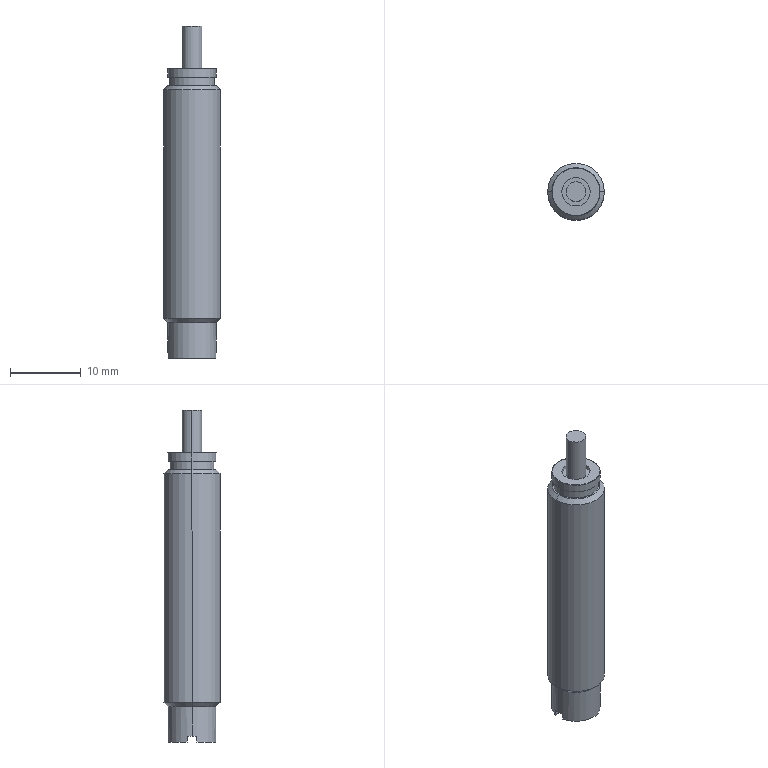Component | SolidWorks | RB0806-1_RB0806-1-1 | 1 solid | 29 faces | box 8 x 8 x 46.8 mm | volume 1959 mm3 | cylinder 12 | plane 11 | cone 4 | spline 2 | commonest cylinder face diameters 6.8 x4 8 x2 6.3 x2 4 x2 2.8 x2
STEP:
#1=COLOUR_RGB('',0.7922,0.8196,0.9333);
#2=FILL_AREA_STYLE_COLOUR('',#1);
#3=FILL_AREA_STYLE('',(#2));
#4=SURFACE_STYLE_FILL_AREA(#3);
#5=SURFACE_SIDE_STYLE('',(#4));
#6=SURFACE_STYLE_USAGE(.BOTH.,#5);
#7=PRESENTATION_STYLE_ASSIGNMENT((#6));
#8=CARTESIAN_POINT('',(-0.9725,1.668,-0.2362));
#9=VERTEX_POINT('',#8);
#10=CARTESIAN_POINT('',(-0.7087,1.668,-0.2362));
#11=VERTEX_POINT('',#10);
#12=CARTESIAN_POINT('',(-0.9725,1.668,-0.2362));
#13=CARTESIAN_POINT('',(-0.9725,1.932,-0.2362));
#14=CARTESIAN_POINT('',(-0.7087,1.932,-0.2362));
#15=CARTESIAN_POINT('',(-0.7087,1.668,-0.2362));
#16=(BOUNDED_CURVE()B_SPLINE_CURVE(3,(#12,#13,#14,#15),.UNSPECIFIED.,.F.,.T.)B_SPLINE_CURVE_WITH_KNOTS((4,4),(0.,1.),.UNSPECIFIED.)CURVE()GEOMETRIC_REPRESENTATION_ITEM()RATIONAL_B_SPLINE_CURVE((1.,0.3333,0.3333,1.))REPRESENTATION_ITEM(''));
#17=EDGE_CURVE('',#9,#11,#16,.T.);
#18=ORIENTED_EDGE('',*,*,#17,.T.);
#19=CARTESIAN_POINT('',(-0.7067,1.668,-0.2382));
#20=VERTEX_POINT('',#19);
#21=CARTESIAN_POINT('',(-0.7087,1.668,-0.2382));
#22=DIRECTION('',(0.,1.,-0.));
#23=DIRECTION('',(1.,0.,0.));
#24=AXIS2_PLACEMENT_3D('',#21,#22,#23);
#25=CIRCLE('',#24,0.001969);
#26=EDGE_CURVE('',#11,#20,#25,.T.);
#27=ORIENTED_EDGE('',*,*,#26,.T.);
#28=CARTESIAN_POINT('',(-0.9744,1.668,-0.2382));
#29=VERTEX_POINT('',#28);
#30=CARTESIAN_POINT('',(-0.8406,1.668,-0.2382));
#31=DIRECTION('',(0.,-0.,-1.));
#32=DIRECTION('',(1.,0.,0.));
#33=AXIS2_PLACEMENT_3D('',#30,#31,#32);
#34=CIRCLE('',#33,0.1339);
#35=EDGE_CURVE('',#29,#20,#34,.T.);
#36=ORIENTED_EDGE('',*,*,#35,.F.);
#37=CARTESIAN_POINT('',(-0.9725,1.668,-0.2382));
#38=DIRECTION('',(-0.,-1.,0.));
#39=DIRECTION('',(-1.,0.,0.));
#40=AXIS2_PLACEMENT_3D('',#37,#38,#39);
#41=CIRCLE('',#40,0.001969);
#42=EDGE_CURVE('',#9,#29,#41,.T.);
#43=ORIENTED_EDGE('',*,*,#42,.F.);
#44=EDGE_LOOP('',(#18,#27,#36,#43));
#45=FACE_OUTER_BOUND('',#44,.T.);
#46=CARTESIAN_POINT('',(-0.7087,1.668,-0.2362));
#47=CARTESIAN_POINT('',(-0.7087,1.932,-0.2362));
#48=CARTESIAN_POINT('',(-0.9725,1.932,-0.2362));
#49=CARTESIAN_POINT('',(-0.9725,1.668,-0.2362));
#50=CARTESIAN_POINT('',(-0.7075,1.668,-0.2362));
#51=CARTESIAN_POINT('',(-0.7075,1.934,-0.2362));
#52=CARTESIAN_POINT('',(-0.9736,1.934,-0.2362));
#53=CARTESIAN_POINT('',(-0.9736,1.668,-0.2362));
#54=CARTESIAN_POINT('',(-0.7067,1.668,-0.237));
#55=CARTESIAN_POINT('',(-0.7067,1.936,-0.237));
#56=CARTESIAN_POINT('',(-0.9744,1.936,-0.237));
#57=CARTESIAN_POINT('',(-0.9744,1.668,-0.237));
#58=CARTESIAN_POINT('',(-0.7067,1.668,-0.2382));
#59=CARTESIAN_POINT('',(-0.7067,1.936,-0.2382));
#60=CARTESIAN_POINT('',(-0.9744,1.936,-0.2382));
#61=CARTESIAN_POINT('',(-0.9744,1.668,-0.2382));
#62=(BOUNDED_SURFACE()B_SPLINE_SURFACE(3,3,((#46,#47,#48,#49),(#50,#51,#52,#53),(#54,#55,#56,#57),(#58,#59,#60,#61)),.UNSPECIFIED.,.F.,.F.,.F.)B_SPLINE_SURFACE_WITH_KNOTS((4,4),(4,4),(0.,1.),(0.,1.),.UNSPECIFIED.)GEOMETRIC_REPRESENTATION_ITEM()RATIONAL_B_SPLINE_SURFACE(((1.,0.3333,0.3333,1.),(0.8047,0.2682,0.2682,0.8047),(0.8047,0.2682,0.2682,0.8047),(1.,0.3333,0.3333,1.)))REPRESENTATION_ITEM('')SURFACE());
#63=ADVANCED_FACE('',(#45),#62,.T.);
#64=CARTESIAN_POINT('',(-0.6831,1.668,-0.3549));
#65=VERTEX_POINT('',#64);
#66=CARTESIAN_POINT('',(-0.9981,1.668,-0.3549));
#67=VERTEX_POINT('',#66);
#68=CARTESIAN_POINT('',(-0.8406,1.668,-0.3549));
#69=DIRECTION('',(0.,-0.,-1.));
#70=DIRECTION('',(1.,0.,0.));
#71=AXIS2_PLACEMENT_3D('',#68,#69,#70);
#72=CIRCLE('',#71,0.1575);
#73=EDGE_CURVE('',#65,#67,#72,.T.);
#74=ORIENTED_EDGE('',*,*,#73,.T.);
#75=CARTESIAN_POINT('',(-0.9981,1.668,-1.622));
#76=VERTEX_POINT('',#75);
#77=CARTESIAN_POINT('',(-0.9981,1.668,-0.9882));
#78=DIRECTION('',(0.,-0.,-1.));
#79=VECTOR('',#78,39.37);
#80=LINE('',#77,#79);
#81=EDGE_CURVE('',#67,#76,#80,.T.);
#82=ORIENTED_EDGE('',*,*,#81,.T.);
#83=CARTESIAN_POINT('',(-0.6831,1.668,-1.622));
#84=VERTEX_POINT('',#83);
#85=CARTESIAN_POINT('',(-0.8406,1.668,-1.622));
#86=DIRECTION('',(-0.,0.,1.));
#87=DIRECTION('',(1.,0.,0.));
#88=AXIS2_PLACEMENT_3D('',#85,#86,#87);
#89=CIRCLE('',#88,0.1575);
#90=EDGE_CURVE('',#76,#84,#89,.T.);
#91=ORIENTED_EDGE('',*,*,#90,.T.);
#92=CARTESIAN_POINT('',(-0.6831,1.668,-0.9882));
#93=DIRECTION('',(0.,-0.,-1.));
#94=VECTOR('',#93,39.37);
#95=LINE('',#92,#94);
#96=EDGE_CURVE('',#65,#84,#95,.T.);
#97=ORIENTED_EDGE('',*,*,#96,.F.);
#98=EDGE_LOOP('',(#74,#82,#91,#97));
#99=FACE_OUTER_BOUND('',#98,.T.);
#100=CARTESIAN_POINT('',(-0.8406,1.668,-0.9882));
#101=DIRECTION('',(0.,-0.,-1.));
#102=DIRECTION('',(1.,0.,0.));
#103=AXIS2_PLACEMENT_3D('',#100,#101,#102);
#104=CYLINDRICAL_SURFACE('',#103,0.1575);
#105=ADVANCED_FACE('',(#99),#104,.T.);
#106=CARTESIAN_POINT('',(-0.7073,1.668,-0.3307));
#107=VERTEX_POINT('',#106);
#108=CARTESIAN_POINT('',(-0.9739,1.668,-0.3307));
#109=VERTEX_POINT('',#108);
#110=CARTESIAN_POINT('',(-0.8406,1.668,-0.3307));
#111=DIRECTION('',(0.,-0.,-1.));
#112=DIRECTION('',(1.,0.,0.));
#113=AXIS2_PLACEMENT_3D('',#110,#111,#112);
#114=CIRCLE('',#113,0.1333);
#115=EDGE_CURVE('',#107,#109,#114,.T.);
#116=ORIENTED_EDGE('',*,*,#115,.T.);
#117=CARTESIAN_POINT('',(-0.9981,1.668,-0.3549));
#118=DIRECTION('',(-0.7071,-0.,-0.7071));
#119=VECTOR('',#118,39.37);
#120=LINE('',#117,#119);
#121=EDGE_CURVE('',#109,#67,#120,.T.);
#122=ORIENTED_EDGE('',*,*,#121,.T.);
#123=ORIENTED_EDGE('',*,*,#73,.F.);
#124=CARTESIAN_POINT('',(-0.6831,1.668,-0.3549));
#125=DIRECTION('',(0.7071,-0.,-0.7071));
#126=VECTOR('',#125,39.37);
#127=LINE('',#124,#126);
#128=EDGE_CURVE('',#107,#65,#127,.T.);
#129=ORIENTED_EDGE('',*,*,#128,.F.);
#130=EDGE_LOOP('',(#116,#122,#123,#129));
#131=FACE_OUTER_BOUND('',#130,.T.);
#132=CARTESIAN_POINT('',(-0.8406,1.668,-0.3549));
#133=DIRECTION('',(0.,-0.,-1.));
#134=DIRECTION('',(1.,0.,0.));
#135=AXIS2_PLACEMENT_3D('',#132,#133,#134);
#136=CONICAL_SURFACE('',#135,0.1575,0.7854);
#137=ADVANCED_FACE('',(#131),#136,.T.);
#138=CARTESIAN_POINT('',(-0.9739,1.668,-1.646));
#139=VERTEX_POINT('',#138);
#140=CARTESIAN_POINT('',(-0.7073,1.668,-1.646));
#141=VERTEX_POINT('',#140);
#142=CARTESIAN_POINT('',(-0.8406,1.668,-1.646));
#143=DIRECTION('',(-0.,0.,1.));
#144=DIRECTION('',(-1.,0.,0.));
#145=AXIS2_PLACEMENT_3D('',#142,#143,#144);
#146=CIRCLE('',#145,0.1333);
#147=EDGE_CURVE('',#139,#141,#146,.T.);
#148=ORIENTED_EDGE('',*,*,#147,.T.);
#149=CARTESIAN_POINT('',(-0.6831,1.668,-1.622));
#150=DIRECTION('',(0.7071,-0.,0.7071));
#151=VECTOR('',#150,39.37);
#152=LINE('',#149,#151);
#153=EDGE_CURVE('',#141,#84,#152,.T.);
#154=ORIENTED_EDGE('',*,*,#153,.T.);
#155=ORIENTED_EDGE('',*,*,#90,.F.);
#156=CARTESIAN_POINT('',(-0.9981,1.668,-1.622));
#157=DIRECTION('',(-0.7071,0.,0.7071));
#158=VECTOR('',#157,39.37);
#159=LINE('',#156,#158);
#160=EDGE_CURVE('',#139,#76,#159,.T.);
#161=ORIENTED_EDGE('',*,*,#160,.F.);
#162=EDGE_LOOP('',(#148,#154,#155,#161));
#163=FACE_OUTER_BOUND('',#162,.T.);
#164=CARTESIAN_POINT('',(-0.8406,1.668,-1.622));
#165=DIRECTION('',(-0.,0.,1.));
#166=DIRECTION('',(-1.,0.,0.));
#167=AXIS2_PLACEMENT_3D('',#164,#165,#166);
#168=CONICAL_SURFACE('',#167,0.1575,0.7854);
#169=ADVANCED_FACE('',(#163),#168,.T.);
#170=CARTESIAN_POINT('',(-0.7166,1.668,-0.2835));
#171=VERTEX_POINT('',#170);
#172=CARTESIAN_POINT('',(-0.9646,1.668,-0.2835));
#173=VERTEX_POINT('',#172);
#174=CARTESIAN_POINT('',(-0.8406,1.668,-0.2835));
#175=DIRECTION('',(0.,-0.,-1.));
#176=DIRECTION('',(1.,0.,0.));
#177=AXIS2_PLACEMENT_3D('',#174,#175,#176);
#178=CIRCLE('',#177,0.124);
#179=EDGE_CURVE('',#171,#173,#178,.T.);
#180=ORIENTED_EDGE('',*,*,#179,.T.);
#181=CARTESIAN_POINT('',(-0.9646,1.668,-0.3307));
#182=VERTEX_POINT('',#181);
#183=CARTESIAN_POINT('',(-0.9646,1.668,-0.3071));
#184=DIRECTION('',(0.,-0.,-1.));
#185=VECTOR('',#184,39.37);
#186=LINE('',#183,#185);
#187=EDGE_CURVE('',#173,#182,#186,.T.);
#188=ORIENTED_EDGE('',*,*,#187,.T.);
#189=CARTESIAN_POINT('',(-0.7166,1.668,-0.3307));
#190=VERTEX_POINT('',#189);
#191=CARTESIAN_POINT('',(-0.8406,1.668,-0.3307));
#192=DIRECTION('',(0.,-0.,-1.));
#193=DIRECTION('',(1.,0.,0.));
#194=AXIS2_PLACEMENT_3D('',#191,#192,#193);
#195=CIRCLE('',#194,0.124);
#196=EDGE_CURVE('',#190,#182,#195,.T.);
#197=ORIENTED_EDGE('',*,*,#196,.F.);
#198=CARTESIAN_POINT('',(-0.7166,1.668,-0.3071));
#199=DIRECTION('',(0.,-0.,-1.));
#200=VECTOR('',#199,39.37);
#201=LINE('',#198,#200);
#202=EDGE_CURVE('',#171,#190,#201,.T.);
#203=ORIENTED_EDGE('',*,*,#202,.F.);
#204=EDGE_LOOP('',(#180,#188,#197,#203));
#205=FACE_OUTER_BOUND('',#204,.T.);
#206=CARTESIAN_POINT('',(-0.8406,1.668,-0.3071));
#207=DIRECTION('',(0.,-0.,-1.));
#208=DIRECTION('',(1.,0.,0.));
#209=AXIS2_PLACEMENT_3D('',#206,#207,#208);
#210=CYLINDRICAL_SURFACE('',#209,0.124);
#211=ADVANCED_FACE('',(#205),#210,.T.);
#212=CARTESIAN_POINT('',(-0.9744,1.668,-1.646));
#213=VERTEX_POINT('',#212);
#214=CARTESIAN_POINT('',(-0.7067,1.668,-1.646));
#215=VERTEX_POINT('',#214);
#216=CARTESIAN_POINT('',(-0.8406,1.668,-1.646));
#217=DIRECTION('',(-0.,0.,1.));
#218=DIRECTION('',(1.,0.,0.));
#219=AXIS2_PLACEMENT_3D('',#216,#217,#218);
#220=CIRCLE('',#219,0.1339);
#221=EDGE_CURVE('',#213,#215,#220,.T.);
#222=ORIENTED_EDGE('',*,*,#221,.F.);
#223=CARTESIAN_POINT('',(-0.9744,1.668,-1.811));
#224=VERTEX_POINT('',#223);
#225=CARTESIAN_POINT('',(-0.9744,1.668,-1.744));
#226=DIRECTION('',(0.,-0.,-1.));
#227=VECTOR('',#226,39.37);
#228=LINE('',#225,#227);
#229=EDGE_CURVE('',#213,#224,#228,.T.);
#230=ORIENTED_EDGE('',*,*,#229,.T.);
#231=CARTESIAN_POINT('',(-0.9716,1.64,-1.811));
#232=VERTEX_POINT('',#231);
#233=CARTESIAN_POINT('',(-0.8406,1.668,-1.811));
#234=DIRECTION('',(-0.,0.,1.));
#235=DIRECTION('',(1.,0.,0.));
#236=AXIS2_PLACEMENT_3D('',#233,#234,#235);
#237=CIRCLE('',#236,0.1339);
#238=EDGE_CURVE('',#224,#232,#237,.T.);
#239=ORIENTED_EDGE('',*,*,#238,.T.);
#240=CARTESIAN_POINT('',(-0.9716,1.64,-1.843));
#241=VERTEX_POINT('',#240);
#242=CARTESIAN_POINT('',(-0.9716,1.64,-1.843));
#243=DIRECTION('',(0.,-0.,-1.));
#244=VECTOR('',#243,39.37);
#245=LINE('',#242,#244);
#246=EDGE_CURVE('',#232,#241,#245,.T.);
#247=ORIENTED_EDGE('',*,*,#246,.T.);
#248=CARTESIAN_POINT('',(-0.7096,1.64,-1.843));
#249=VERTEX_POINT('',#248);
#250=CARTESIAN_POINT('',(-0.8406,1.668,-1.843));
#251=DIRECTION('',(-0.,0.,1.));
#252=DIRECTION('',(1.,0.,0.));
#253=AXIS2_PLACEMENT_3D('',#250,#251,#252);
#254=CIRCLE('',#253,0.1339);
#255=EDGE_CURVE('',#241,#249,#254,.T.);
#256=ORIENTED_EDGE('',*,*,#255,.T.);
#257=CARTESIAN_POINT('',(-0.7096,1.64,-1.811));
#258=VERTEX_POINT('',#257);
#259=CARTESIAN_POINT('',(-0.7096,1.64,-1.843));
#260=DIRECTION('',(-0.,0.,1.));
#261=VECTOR('',#260,39.37);
#262=LINE('',#259,#261);
#263=EDGE_CURVE('',#249,#258,#262,.T.);
#264=ORIENTED_EDGE('',*,*,#263,.T.);
#265=CARTESIAN_POINT('',(-0.7067,1.668,-1.811));
#266=VERTEX_POINT('',#265);
#267=CARTESIAN_POINT('',(-0.8406,1.668,-1.811));
#268=DIRECTION('',(-0.,0.,1.));
#269=DIRECTION('',(1.,0.,0.));
#270=AXIS2_PLACEMENT_3D('',#267,#268,#269);
#271=CIRCLE('',#270,0.1339);
#272=EDGE_CURVE('',#258,#266,#271,.T.);
#273=ORIENTED_EDGE('',*,*,#272,.T.);
#274=CARTESIAN_POINT('',(-0.7067,1.668,-1.744));
#275=DIRECTION('',(0.,-0.,-1.));
#276=VECTOR('',#275,39.37);
#277=LINE('',#274,#276);
#278=EDGE_CURVE('',#215,#266,#277,.T.);
#279=ORIENTED_EDGE('',*,*,#278,.F.);
#280=EDGE_LOOP('',(#222,#230,#239,#247,#256,#264,#273,#279));
#281=FACE_OUTER_BOUND('',#280,.T.);
#282=CARTESIAN_POINT('',(-0.8406,1.668,-1.744));
#283=DIRECTION('',(0.,-0.,-1.));
#284=DIRECTION('',(1.,0.,0.));
#285=AXIS2_PLACEMENT_3D('',#282,#283,#284);
#286=CYLINDRICAL_SURFACE('',#285,0.1339);
#287=ADVANCED_FACE('',(#281),#286,.T.);
#288=CARTESIAN_POINT('',(-0.8406,1.668,-0.2382));
#289=DIRECTION('',(0.,-0.,-1.));
#290=DIRECTION('',(1.,0.,0.));
#291=AXIS2_PLACEMENT_3D('',#288,#289,#290);
#292=CIRCLE('',#291,0.1339);
#293=EDGE_CURVE('',#20,#29,#292,.T.);
#294=ORIENTED_EDGE('',*,*,#293,.T.);
#295=CARTESIAN_POINT('',(-0.9744,1.668,-0.2835));
#296=VERTEX_POINT('',#295);
#297=CARTESIAN_POINT('',(-0.9744,1.668,-0.2608));
#298=DIRECTION('',(0.,-0.,-1.));
#299=VECTOR('',#298,39.37);
#300=LINE('',#297,#299);
#301=EDGE_CURVE('',#29,#296,#300,.T.);
#302=ORIENTED_EDGE('',*,*,#301,.T.);
#303=CARTESIAN_POINT('',(-0.7067,1.668,-0.2835));
#304=VERTEX_POINT('',#303);
#305=CARTESIAN_POINT('',(-0.8406,1.668,-0.2835));
#306=DIRECTION('',(0.,-0.,-1.));
#307=DIRECTION('',(1.,0.,0.));
#308=AXIS2_PLACEMENT_3D('',#305,#306,#307);
#309=CIRCLE('',#308,0.1339);
#310=EDGE_CURVE('',#304,#296,#309,.T.);
#311=ORIENTED_EDGE('',*,*,#310,.F.);
#312=CARTESIAN_POINT('',(-0.7067,1.668,-0.2608));
#313=DIRECTION('',(0.,-0.,-1.));
#314=VECTOR('',#313,39.37);
#315=LINE('',#312,#314);
#316=EDGE_CURVE('',#20,#304,#315,.T.);
#317=ORIENTED_EDGE('',*,*,#316,.F.);
#318=EDGE_LOOP('',(#294,#302,#311,#317));
#319=FACE_OUTER_BOUND('',#318,.T.);
#320=CARTESIAN_POINT('',(-0.8406,1.668,-0.2608));
#321=DIRECTION('',(0.,-0.,-1.));
#322=DIRECTION('',(1.,0.,0.));
#323=AXIS2_PLACEMENT_3D('',#320,#321,#322);
#324=CYLINDRICAL_SURFACE('',#323,0.1339);
#325=ADVANCED_FACE('',(#319),#324,.T.);
#326=CARTESIAN_POINT('',(-0.7618,1.668,-0.2559));
#327=VERTEX_POINT('',#326);
#328=CARTESIAN_POINT('',(-0.9193,1.668,-0.2559));
#329=VERTEX_POINT('',#328);
#330=CARTESIAN_POINT('',(-0.8406,1.668,-0.2559));
#331=DIRECTION('',(-0.,0.,1.));
#332=DIRECTION('',(-1.,0.,0.));
#333=AXIS2_PLACEMENT_3D('',#330,#331,#332);
#334=CIRCLE('',#333,0.07874);
#335=EDGE_CURVE('',#327,#329,#334,.T.);
#336=ORIENTED_EDGE('',*,*,#335,.F.);
#337=CARTESIAN_POINT('',(-0.7618,1.668,-0.2362));
#338=VERTEX_POINT('',#337);
#339=CARTESIAN_POINT('',(-0.7618,1.668,-0.2362));
#340=DIRECTION('',(-0.,0.,1.));
#341=VECTOR('',#340,39.37);
#342=LINE('',#339,#341);
#343=EDGE_CURVE('',#327,#338,#342,.T.);
#344=ORIENTED_EDGE('',*,*,#343,.T.);
#345=CARTESIAN_POINT('',(-0.9193,1.668,-0.2362));
#346=VERTEX_POINT('',#345);
#347=CARTESIAN_POINT('',(-0.8406,1.668,-0.2362));
#348=DIRECTION('',(0.,-0.,-1.));
#349=DIRECTION('',(-1.,0.,0.));
#350=AXIS2_PLACEMENT_3D('',#347,#348,#349);
#351=CIRCLE('',#350,0.07874);
#352=EDGE_CURVE('',#346,#338,#351,.T.);
#353=ORIENTED_EDGE('',*,*,#352,.F.);
#354=CARTESIAN_POINT('',(-0.9193,1.668,-0.2362));
#355=DIRECTION('',(-0.,0.,1.));
#356=VECTOR('',#355,39.37);
#357=LINE('',#354,#356);
#358=EDGE_CURVE('',#329,#346,#357,.T.);
#359=ORIENTED_EDGE('',*,*,#358,.F.);
#360=EDGE_LOOP('',(#336,#344,#353,#359));
#361=FACE_OUTER_BOUND('',#360,.T.);
#362=CARTESIAN_POINT('',(-0.8406,1.668,-0.2362));
#363=DIRECTION('',(-0.,0.,1.));
#364=DIRECTION('',(-1.,0.,0.));
#365=AXIS2_PLACEMENT_3D('',#362,#363,#364);
#366=CYLINDRICAL_SURFACE('',#365,0.07874);
#367=ADVANCED_FACE('',(#361),#366,.F.);
#368=CARTESIAN_POINT('',(-0.7855,1.668,-0.));
#369=VERTEX_POINT('',#368);
#370=CARTESIAN_POINT('',(-0.8957,1.668,-0.));
#371=VERTEX_POINT('',#370);
#372=CARTESIAN_POINT('',(-0.8406,1.668,-0.));
#373=DIRECTION('',(0.,-0.,-1.));
#374=DIRECTION('',(1.,0.,0.));
#375=AXIS2_PLACEMENT_3D('',#372,#373,#374);
#376=CIRCLE('',#375,0.05512);
#377=EDGE_CURVE('',#369,#371,#376,.T.);
#378=ORIENTED_EDGE('',*,*,#377,.T.);
#379=CARTESIAN_POINT('',(-0.8957,1.668,-0.2559));
#380=VERTEX_POINT('',#379);
#381=CARTESIAN_POINT('',(-0.8957,1.668,-0.2362));
#382=DIRECTION('',(0.,-0.,-1.));
#383=VECTOR('',#382,39.37);
#384=LINE('',#381,#383);
#385=EDGE_CURVE('',#371,#380,#384,.T.);
#386=ORIENTED_EDGE('',*,*,#385,.T.);
#387=CARTESIAN_POINT('',(-0.7855,1.668,-0.2559));
#388=VERTEX_POINT('',#387);
#389=CARTESIAN_POINT('',(-0.8406,1.668,-0.2559));
#390=DIRECTION('',(-0.,0.,1.));
#391=DIRECTION('',(1.,0.,0.));
#392=AXIS2_PLACEMENT_3D('',#389,#390,#391);
#393=CIRCLE('',#392,0.05512);
#394=EDGE_CURVE('',#380,#388,#393,.T.);
#395=ORIENTED_EDGE('',*,*,#394,.T.);
#396=CARTESIAN_POINT('',(-0.7855,1.668,-0.2362));
#397=DIRECTION('',(0.,-0.,-1.));
#398=VECTOR('',#397,39.37);
#399=LINE('',#396,#398);
#400=EDGE_CURVE('',#369,#388,#399,.T.);
#401=ORIENTED_EDGE('',*,*,#400,.F.);
#402=EDGE_LOOP('',(#378,#386,#395,#401));
#403=FACE_OUTER_BOUND('',#402,.T.);
#404=CARTESIAN_POINT('',(-0.8406,1.668,-0.2362));
#405=DIRECTION('',(0.,-0.,-1.));
#406=DIRECTION('',(1.,0.,0.));
#407=AXIS2_PLACEMENT_3D('',#404,#405,#406);
#408=CYLINDRICAL_SURFACE('',#407,0.05512);
#409=ADVANCED_FACE('',(#403),#408,.T.);
#410=ORIENTED_EDGE('',*,*,#81,.F.);
#411=CARTESIAN_POINT('',(-0.8406,1.668,-0.3549));
#412=DIRECTION('',(0.,-0.,-1.));
#413=DIRECTION('',(1.,0.,0.));
#414=AXIS2_PLACEMENT_3D('',#411,#412,#413);
#415=CIRCLE('',#414,0.1575);
#416=EDGE_CURVE('',#67,#65,#415,.T.);
#417=ORIENTED_EDGE('',*,*,#416,.T.);
#418=ORIENTED_EDGE('',*,*,#96,.T.);
#419=CARTESIAN_POINT('',(-0.8406,1.668,-1.622));
#420=DIRECTION('',(-0.,0.,1.));
#421=DIRECTION('',(1.,0.,0.));
#422=AXIS2_PLACEMENT_3D('',#419,#420,#421);
#423=CIRCLE('',#422,0.1575);
#424=EDGE_CURVE('',#84,#76,#423,.T.);
#425=ORIENTED_EDGE('',*,*,#424,.T.);
#426=EDGE_LOOP('',(#410,#417,#418,#425));
#427=FACE_OUTER_BOUND('',#426,.T.);
#428=CARTESIAN_POINT('',(-0.8406,1.668,-0.9882));
#429=DIRECTION('',(0.,-0.,-1.));
#430=DIRECTION('',(1.,0.,0.));
#431=AXIS2_PLACEMENT_3D('',#428,#429,#430);
#432=CYLINDRICAL_SURFACE('',#431,0.1575);
#433=ADVANCED_FACE('',(#427),#432,.T.);
#434=ORIENTED_EDGE('',*,*,#121,.F.);
#435=CARTESIAN_POINT('',(-0.8406,1.668,-0.3307));
#436=DIRECTION('',(0.,-0.,-1.));
#437=DIRECTION('',(1.,0.,0.));
#438=AXIS2_PLACEMENT_3D('',#435,#436,#437);
#439=CIRCLE('',#438,0.1333);
#440=EDGE_CURVE('',#109,#107,#439,.T.);
#441=ORIENTED_EDGE('',*,*,#440,.T.);
#442=ORIENTED_EDGE('',*,*,#128,.T.);
#443=ORIENTED_EDGE('',*,*,#416,.F.);
#444=EDGE_LOOP('',(#434,#441,#442,#443));
#445=FACE_OUTER_BOUND('',#444,.T.);
#446=CARTESIAN_POINT('',(-0.8406,1.668,-0.3549));
#447=DIRECTION('',(0.,-0.,-1.));
#448=DIRECTION('',(1.,0.,0.));
#449=AXIS2_PLACEMENT_3D('',#446,#447,#448);
#450=CONICAL_SURFACE('',#449,0.1575,0.7854);
#451=ADVANCED_FACE('',(#445),#450,.T.);
#452=ORIENTED_EDGE('',*,*,#153,.F.);
#453=CARTESIAN_POINT('',(-0.8406,1.668,-1.646));
#454=DIRECTION('',(-0.,0.,1.));
#455=DIRECTION('',(-1.,0.,0.));
#456=AXIS2_PLACEMENT_3D('',#453,#454,#455);
#457=CIRCLE('',#456,0.1333);
#458=EDGE_CURVE('',#141,#139,#457,.T.);
#459=ORIENTED_EDGE('',*,*,#458,.T.);
#460=ORIENTED_EDGE('',*,*,#160,.T.);
#461=ORIENTED_EDGE('',*,*,#424,.F.);
#462=EDGE_LOOP('',(#452,#459,#460,#461));
#463=FACE_OUTER_BOUND('',#462,.T.);
#464=CARTESIAN_POINT('',(-0.8406,1.668,-1.622));
#465=DIRECTION('',(-0.,0.,1.));
#466=DIRECTION('',(-1.,0.,0.));
#467=AXIS2_PLACEMENT_3D('',#464,#465,#466);
#468=CONICAL_SURFACE('',#467,0.1575,0.7854);
#469=ADVANCED_FACE('',(#463),#468,.T.);
#470=ORIENTED_EDGE('',*,*,#115,.F.);
#471=ORIENTED_EDGE('',*,*,#440,.F.);
#472=EDGE_LOOP('',(#470,#471));
#473=FACE_OUTER_BOUND('',#472,.T.);
#474=ORIENTED_EDGE('',*,*,#196,.T.);
#475=CARTESIAN_POINT('',(-0.8406,1.668,-0.3307));
#476=DIRECTION('',(0.,-0.,-1.));
#477=DIRECTION('',(1.,0.,0.));
#478=AXIS2_PLACEMENT_3D('',#475,#476,#477);
#479=CIRCLE('',#478,0.124);
#480=EDGE_CURVE('',#182,#190,#479,.T.);
#481=ORIENTED_EDGE('',*,*,#480,.T.);
#482=EDGE_LOOP('',(#474,#481));
#483=FACE_BOUND('',#482,.T.);
#484=CARTESIAN_POINT('',(-0.8406,1.539,-0.3307));
#485=DIRECTION('',(-0.,0.,1.));
#486=DIRECTION('',(-1.,0.,-0.));
#487=AXIS2_PLACEMENT_3D('',#484,#485,#486);
#488=PLANE('',#487);
#489=ADVANCED_FACE('',(#473,#483),#488,.T.);
#490=CARTESIAN_POINT('',(-0.8406,1.668,-1.646));
#491=DIRECTION('',(-0.,0.,1.));
#492=DIRECTION('',(1.,0.,0.));
#493=AXIS2_PLACEMENT_3D('',#490,#491,#492);
#494=CIRCLE('',#493,0.1339);
#495=EDGE_CURVE('',#215,#213,#494,.T.);
#496=ORIENTED_EDGE('',*,*,#495,.T.);
#497=ORIENTED_EDGE('',*,*,#221,.T.);
#498=EDGE_LOOP('',(#496,#497));
#499=FACE_OUTER_BOUND('',#498,.T.);
#500=ORIENTED_EDGE('',*,*,#147,.F.);
#501=ORIENTED_EDGE('',*,*,#458,.F.);
#502=EDGE_LOOP('',(#500,#501));
#503=FACE_BOUND('',#502,.T.);
#504=CARTESIAN_POINT('',(-0.8406,1.534,-1.646));
#505=DIRECTION('',(-0.,0.,1.));
#506=DIRECTION('',(-1.,0.,-0.));
#507=AXIS2_PLACEMENT_3D('',#504,#505,#506);
#508=PLANE('',#507);
#509=ADVANCED_FACE('',(#499,#503),#508,.T.);
#510=ORIENTED_EDGE('',*,*,#187,.F.);
#511=CARTESIAN_POINT('',(-0.8406,1.668,-0.2835));
#512=DIRECTION('',(0.,-0.,-1.));
#513=DIRECTION('',(1.,0.,0.));
#514=AXIS2_PLACEMENT_3D('',#511,#512,#513);
#515=CIRCLE('',#514,0.124);
#516=EDGE_CURVE('',#173,#171,#515,.T.);
#517=ORIENTED_EDGE('',*,*,#516,.T.);
#518=ORIENTED_EDGE('',*,*,#202,.T.);
#519=ORIENTED_EDGE('',*,*,#480,.F.);
#520=EDGE_LOOP('',(#510,#517,#518,#519));
#521=FACE_OUTER_BOUND('',#520,.T.);
#522=CARTESIAN_POINT('',(-0.8406,1.668,-0.3071));
#523=DIRECTION('',(0.,-0.,-1.));
#524=DIRECTION('',(1.,0.,0.));
#525=AXIS2_PLACEMENT_3D('',#522,#523,#524);
#526=CYLINDRICAL_SURFACE('',#525,0.124);
#527=ADVANCED_FACE('',(#521),#526,.T.);
#528=ORIENTED_EDGE('',*,*,#229,.F.);
#529=ORIENTED_EDGE('',*,*,#495,.F.);
#530=ORIENTED_EDGE('',*,*,#278,.T.);
#531=CARTESIAN_POINT('',(-0.7096,1.695,-1.811));
#532=VERTEX_POINT('',#531);
#533=CARTESIAN_POINT('',(-0.8406,1.668,-1.811));
#534=DIRECTION('',(-0.,0.,1.));
#535=DIRECTION('',(1.,0.,0.));
#536=AXIS2_PLACEMENT_3D('',#533,#534,#535);
#537=CIRCLE('',#536,0.1339);
#538=EDGE_CURVE('',#266,#532,#537,.T.);
#539=ORIENTED_EDGE('',*,*,#538,.T.);
#540=CARTESIAN_POINT('',(-0.7096,1.695,-1.843));
#541=VERTEX_POINT('',#540);
#542=CARTESIAN_POINT('',(-0.7096,1.695,-1.811));
#543=DIRECTION('',(0.,-0.,-1.));
#544=VECTOR('',#543,39.37);
#545=LINE('',#542,#544);
#546=EDGE_CURVE('',#532,#541,#545,.T.);
#547=ORIENTED_EDGE('',*,*,#546,.T.);
#548=CARTESIAN_POINT('',(-0.9716,1.695,-1.843));
#549=VERTEX_POINT('',#548);
#550=CARTESIAN_POINT('',(-0.8406,1.668,-1.843));
#551=DIRECTION('',(-0.,0.,1.));
#552=DIRECTION('',(1.,0.,0.));
#553=AXIS2_PLACEMENT_3D('',#550,#551,#552);
#554=CIRCLE('',#553,0.1339);
#555=EDGE_CURVE('',#541,#549,#554,.T.);
#556=ORIENTED_EDGE('',*,*,#555,.T.);
#557=CARTESIAN_POINT('',(-0.9716,1.695,-1.811));
#558=VERTEX_POINT('',#557);
#559=CARTESIAN_POINT('',(-0.9716,1.695,-1.811));
#560=DIRECTION('',(-0.,0.,1.));
#561=VECTOR('',#560,39.37);
#562=LINE('',#559,#561);
#563=EDGE_CURVE('',#549,#558,#562,.T.);
#564=ORIENTED_EDGE('',*,*,#563,.T.);
#565=CARTESIAN_POINT('',(-0.8406,1.668,-1.811));
#566=DIRECTION('',(-0.,0.,1.));
#567=DIRECTION('',(1.,0.,0.));
#568=AXIS2_PLACEMENT_3D('',#565,#566,#567);
#569=CIRCLE('',#568,0.1339);
#570=EDGE_CURVE('',#558,#224,#569,.T.);
#571=ORIENTED_EDGE('',*,*,#570,.T.);
#572=EDGE_LOOP('',(#528,#529,#530,#539,#547,#556,#564,#571));
#573=FACE_OUTER_BOUND('',#572,.T.);
#574=CARTESIAN_POINT('',(-0.8406,1.668,-1.744));
#575=DIRECTION('',(0.,-0.,-1.));
#576=DIRECTION('',(1.,0.,0.));
#577=AXIS2_PLACEMENT_3D('',#574,#575,#576);
#578=CYLINDRICAL_SURFACE('',#577,0.1339);
#579=ADVANCED_FACE('',(#573),#578,.T.);
#580=ORIENTED_EDGE('',*,*,#179,.F.);
#581=ORIENTED_EDGE('',*,*,#516,.F.);
#582=EDGE_LOOP('',(#580,#581));
#583=FACE_BOUND('',#582,.T.);
#584=ORIENTED_EDGE('',*,*,#310,.T.);
#585=CARTESIAN_POINT('',(-0.8406,1.668,-0.2835));
#586=DIRECTION('',(0.,-0.,-1.));
#587=DIRECTION('',(1.,0.,0.));
#588=AXIS2_PLACEMENT_3D('',#585,#586,#587);
#589=CIRCLE('',#588,0.1339);
#590=EDGE_CURVE('',#296,#304,#589,.T.);
#591=ORIENTED_EDGE('',*,*,#590,.T.);
#592=EDGE_LOOP('',(#584,#591));
#593=FACE_OUTER_BOUND('',#592,.T.);
#594=CARTESIAN_POINT('',(-0.8406,1.539,-0.2835));
#595=DIRECTION('',(0.,-0.,-1.));
#596=DIRECTION('',(1.,-0.,0.));
#597=AXIS2_PLACEMENT_3D('',#594,#595,#596);
#598=PLANE('',#597);
#599=ADVANCED_FACE('',(#583,#593),#598,.T.);
#600=CARTESIAN_POINT('',(-0.8406,1.64,-1.843));
#601=DIRECTION('',(1.,-0.,0.));
#602=VECTOR('',#601,39.37);
#603=LINE('',#600,#602);
#604=EDGE_CURVE('',#241,#249,#603,.T.);
#605=ORIENTED_EDGE('',*,*,#604,.T.);
#606=ORIENTED_EDGE('',*,*,#255,.F.);
#607=EDGE_LOOP('',(#605,#606));
#608=FACE_OUTER_BOUND('',#607,.T.);
#609=CARTESIAN_POINT('',(-0.8406,1.601,-1.843));
#610=DIRECTION('',(0.,-0.,-1.));
#611=DIRECTION('',(1.,-0.,0.));
#612=AXIS2_PLACEMENT_3D('',#609,#610,#611);
#613=PLANE('',#612);
#614=ADVANCED_FACE('',(#608),#613,.T.);
#615=ORIENTED_EDGE('',*,*,#555,.F.);
#616=CARTESIAN_POINT('',(-0.8406,1.695,-1.843));
#617=DIRECTION('',(-1.,0.,-0.));
#618=VECTOR('',#617,39.37);
#619=LINE('',#616,#618);
#620=EDGE_CURVE('',#541,#549,#619,.T.);
#621=ORIENTED_EDGE('',*,*,#620,.T.);
#622=EDGE_LOOP('',(#615,#621));
#623=FACE_OUTER_BOUND('',#622,.T.);
#624=CARTESIAN_POINT('',(-0.8406,1.601,-1.843));
#625=DIRECTION('',(0.,-0.,-1.));
#626=DIRECTION('',(1.,-0.,0.));
#627=AXIS2_PLACEMENT_3D('',#624,#625,#626);
#628=PLANE('',#627);
#629=ADVANCED_FACE('',(#623),#628,.T.);
#630=ORIENTED_EDGE('',*,*,#301,.F.);
#631=ORIENTED_EDGE('',*,*,#35,.T.);
#632=ORIENTED_EDGE('',*,*,#316,.T.);
#633=ORIENTED_EDGE('',*,*,#590,.F.);
#634=EDGE_LOOP('',(#630,#631,#632,#633));
#635=FACE_OUTER_BOUND('',#634,.T.);
#636=CARTESIAN_POINT('',(-0.8406,1.668,-0.2608));
#637=DIRECTION('',(0.,-0.,-1.));
#638=DIRECTION('',(1.,0.,0.));
#639=AXIS2_PLACEMENT_3D('',#636,#637,#638);
#640=CYLINDRICAL_SURFACE('',#639,0.1339);
#641=ADVANCED_FACE('',(#635),#640,.T.);
#642=CARTESIAN_POINT('',(-1.108,1.64,-1.811));
#643=DIRECTION('',(-1.,0.,-0.));
#644=VECTOR('',#643,39.37);
#645=LINE('',#642,#644);
#646=EDGE_CURVE('',#258,#232,#645,.T.);
#647=ORIENTED_EDGE('',*,*,#646,.F.);
#648=ORIENTED_EDGE('',*,*,#263,.F.);
#649=ORIENTED_EDGE('',*,*,#604,.F.);
#650=ORIENTED_EDGE('',*,*,#246,.F.);
#651=EDGE_LOOP('',(#647,#648,#649,#650));
#652=FACE_OUTER_BOUND('',#651,.T.);
#653=CARTESIAN_POINT('',(-1.108,1.64,-1.843));
#654=DIRECTION('',(-0.,-1.,0.));
#655=DIRECTION('',(-1.,0.,-0.));
#656=AXIS2_PLACEMENT_3D('',#653,#654,#655);
#657=PLANE('',#656);
#658=ADVANCED_FACE('',(#652),#657,.F.);
#659=ORIENTED_EDGE('',*,*,#620,.F.);
#660=ORIENTED_EDGE('',*,*,#546,.F.);
#661=CARTESIAN_POINT('',(-1.108,1.695,-1.811));
#662=DIRECTION('',(1.,-0.,0.));
#663=VECTOR('',#662,39.37);
#664=LINE('',#661,#663);
#665=EDGE_CURVE('',#558,#532,#664,.T.);
#666=ORIENTED_EDGE('',*,*,#665,.F.);
#667=ORIENTED_EDGE('',*,*,#563,.F.);
#668=EDGE_LOOP('',(#659,#660,#666,#667));
#669=FACE_OUTER_BOUND('',#668,.T.);
#670=CARTESIAN_POINT('',(-1.108,1.695,-1.811));
#671=DIRECTION('',(0.,1.,-0.));
#672=DIRECTION('',(1.,-0.,0.));
#673=AXIS2_PLACEMENT_3D('',#670,#671,#672);
#674=PLANE('',#673);
#675=ADVANCED_FACE('',(#669),#674,.F.);
#676=ORIENTED_EDGE('',*,*,#26,.F.);
#677=CARTESIAN_POINT('',(-0.8406,1.536,-0.2362));
#678=VERTEX_POINT('',#677);
#679=CARTESIAN_POINT('',(-0.7087,1.668,-0.2362));
#680=CARTESIAN_POINT('',(-0.7087,1.591,-0.2362));
#681=CARTESIAN_POINT('',(-0.7633,1.536,-0.2362));
#682=CARTESIAN_POINT('',(-0.8406,1.536,-0.2362));
#683=(BOUNDED_CURVE()B_SPLINE_CURVE(3,(#679,#680,#681,#682),.UNSPECIFIED.,.F.,.F.)B_SPLINE_CURVE_WITH_KNOTS((4,4),(0.,1.),.UNSPECIFIED.)CURVE()GEOMETRIC_REPRESENTATION_ITEM()RATIONAL_B_SPLINE_CURVE((1.,0.8047,0.8047,1.))REPRESENTATION_ITEM(''));
#684=EDGE_CURVE('',#11,#678,#683,.T.);
#685=ORIENTED_EDGE('',*,*,#684,.T.);
#686=CARTESIAN_POINT('',(-0.8406,1.536,-0.2362));
#687=CARTESIAN_POINT('',(-0.9178,1.536,-0.2362));
#688=CARTESIAN_POINT('',(-0.9725,1.591,-0.2362));
#689=CARTESIAN_POINT('',(-0.9725,1.668,-0.2362));
#690=(BOUNDED_CURVE()B_SPLINE_CURVE(3,(#686,#687,#688,#689),.UNSPECIFIED.,.F.,.F.)B_SPLINE_CURVE_WITH_KNOTS((4,4),(0.,1.),.UNSPECIFIED.)CURVE()GEOMETRIC_REPRESENTATION_ITEM()RATIONAL_B_SPLINE_CURVE((1.,0.8047,0.8047,1.))REPRESENTATION_ITEM(''));
#691=EDGE_CURVE('',#678,#9,#690,.T.);
#692=ORIENTED_EDGE('',*,*,#691,.T.);
#693=ORIENTED_EDGE('',*,*,#42,.T.);
#694=ORIENTED_EDGE('',*,*,#293,.F.);
#695=EDGE_LOOP('',(#676,#685,#692,#693,#694));
#696=FACE_OUTER_BOUND('',#695,.T.);
#697=CARTESIAN_POINT('',(-0.9725,1.668,-0.2362));
#698=CARTESIAN_POINT('',(-0.9725,1.404,-0.2362));
#699=CARTESIAN_POINT('',(-0.7087,1.404,-0.2362));
#700=CARTESIAN_POINT('',(-0.7087,1.668,-0.2362));
#701=CARTESIAN_POINT('',(-0.9736,1.668,-0.2362));
#702=CARTESIAN_POINT('',(-0.9736,1.402,-0.2362));
#703=CARTESIAN_POINT('',(-0.7075,1.402,-0.2362));
#704=CARTESIAN_POINT('',(-0.7075,1.668,-0.2362));
#705=CARTESIAN_POINT('',(-0.9744,1.668,-0.237));
#706=CARTESIAN_POINT('',(-0.9744,1.4,-0.237));
#707=CARTESIAN_POINT('',(-0.7067,1.4,-0.237));
#708=CARTESIAN_POINT('',(-0.7067,1.668,-0.237));
#709=CARTESIAN_POINT('',(-0.9744,1.668,-0.2382));
#710=CARTESIAN_POINT('',(-0.9744,1.4,-0.2382));
#711=CARTESIAN_POINT('',(-0.7067,1.4,-0.2382));
#712=CARTESIAN_POINT('',(-0.7067,1.668,-0.2382));
#713=(BOUNDED_SURFACE()B_SPLINE_SURFACE(3,3,((#697,#698,#699,#700),(#701,#702,#703,#704),(#705,#706,#707,#708),(#709,#710,#711,#712)),.UNSPECIFIED.,.F.,.F.,.F.)B_SPLINE_SURFACE_WITH_KNOTS((4,4),(4,4),(0.,1.),(0.,1.),.UNSPECIFIED.)GEOMETRIC_REPRESENTATION_ITEM()RATIONAL_B_SPLINE_SURFACE(((1.,0.3333,0.3333,1.),(0.8047,0.2682,0.2682,0.8047),(0.8047,0.2682,0.2682,0.8047),(1.,0.3333,0.3333,1.)))REPRESENTATION_ITEM('')SURFACE());
#714=ADVANCED_FACE('',(#696),#713,.T.);
#715=ORIENTED_EDGE('',*,*,#665,.T.);
#716=ORIENTED_EDGE('',*,*,#538,.F.);
#717=ORIENTED_EDGE('',*,*,#272,.F.);
#718=ORIENTED_EDGE('',*,*,#646,.T.);
#719=ORIENTED_EDGE('',*,*,#238,.F.);
#720=ORIENTED_EDGE('',*,*,#570,.F.);
#721=EDGE_LOOP('',(#715,#716,#717,#718,#719,#720));
#722=FACE_OUTER_BOUND('',#721,.T.);
#723=CARTESIAN_POINT('',(-1.108,1.64,-1.811));
#724=DIRECTION('',(-0.,0.,1.));
#725=DIRECTION('',(-1.,0.,-0.));
#726=AXIS2_PLACEMENT_3D('',#723,#724,#725);
#727=PLANE('',#726);
#728=ADVANCED_FACE('',(#722),#727,.F.);
#729=ORIENTED_EDGE('',*,*,#17,.F.);
#730=ORIENTED_EDGE('',*,*,#691,.F.);
#731=ORIENTED_EDGE('',*,*,#684,.F.);
#732=EDGE_LOOP('',(#729,#730,#731));
#733=FACE_OUTER_BOUND('',#732,.T.);
#734=ORIENTED_EDGE('',*,*,#352,.T.);
#735=CARTESIAN_POINT('',(-0.8406,1.668,-0.2362));
#736=DIRECTION('',(0.,-0.,-1.));
#737=DIRECTION('',(-1.,0.,0.));
#738=AXIS2_PLACEMENT_3D('',#735,#736,#737);
#739=CIRCLE('',#738,0.07874);
#740=EDGE_CURVE('',#338,#346,#739,.T.);
#741=ORIENTED_EDGE('',*,*,#740,.T.);
#742=EDGE_LOOP('',(#734,#741));
#743=FACE_BOUND('',#742,.T.);
#744=CARTESIAN_POINT('',(-0.8406,1.602,-0.2362));
#745=DIRECTION('',(-0.,0.,1.));
#746=DIRECTION('',(-1.,0.,-0.));
#747=AXIS2_PLACEMENT_3D('',#744,#745,#746);
#748=PLANE('',#747);
#749=ADVANCED_FACE('',(#733,#743),#748,.T.);
#750=ORIENTED_EDGE('',*,*,#343,.F.);
#751=CARTESIAN_POINT('',(-0.8406,1.668,-0.2559));
#752=DIRECTION('',(-0.,0.,1.));
#753=DIRECTION('',(-1.,0.,0.));
#754=AXIS2_PLACEMENT_3D('',#751,#752,#753);
#755=CIRCLE('',#754,0.07874);
#756=EDGE_CURVE('',#329,#327,#755,.T.);
#757=ORIENTED_EDGE('',*,*,#756,.F.);
#758=ORIENTED_EDGE('',*,*,#358,.T.);
#759=ORIENTED_EDGE('',*,*,#740,.F.);
#760=EDGE_LOOP('',(#750,#757,#758,#759));
#761=FACE_OUTER_BOUND('',#760,.T.);
#762=CARTESIAN_POINT('',(-0.8406,1.668,-0.2362));
#763=DIRECTION('',(-0.,0.,1.));
#764=DIRECTION('',(-1.,0.,0.));
#765=AXIS2_PLACEMENT_3D('',#762,#763,#764);
#766=CYLINDRICAL_SURFACE('',#765,0.07874);
#767=ADVANCED_FACE('',(#761),#766,.F.);
#768=CARTESIAN_POINT('',(-0.8406,1.668,-0.2559));
#769=DIRECTION('',(-0.,0.,1.));
#770=DIRECTION('',(1.,0.,0.));
#771=AXIS2_PLACEMENT_3D('',#768,#769,#770);
#772=CIRCLE('',#771,0.05512);
#773=EDGE_CURVE('',#388,#380,#772,.T.);
#774=ORIENTED_EDGE('',*,*,#773,.F.);
#775=ORIENTED_EDGE('',*,*,#394,.F.);
#776=EDGE_LOOP('',(#774,#775));
#777=FACE_BOUND('',#776,.T.);
#778=ORIENTED_EDGE('',*,*,#756,.T.);
#779=ORIENTED_EDGE('',*,*,#335,.T.);
#780=EDGE_LOOP('',(#778,#779));
#781=FACE_OUTER_BOUND('',#780,.T.);
#782=CARTESIAN_POINT('',(-0.8406,1.668,-0.2559));
#783=DIRECTION('',(0.,-0.,-1.));
#784=DIRECTION('',(1.,-0.,0.));
#785=AXIS2_PLACEMENT_3D('',#782,#783,#784);
#786=PLANE('',#785);
#787=ADVANCED_FACE('',(#777,#781),#786,.F.);
#788=ORIENTED_EDGE('',*,*,#385,.F.);
#789=CARTESIAN_POINT('',(-0.8406,1.668,-0.));
#790=DIRECTION('',(0.,-0.,-1.));
#791=DIRECTION('',(1.,0.,0.));
#792=AXIS2_PLACEMENT_3D('',#789,#790,#791);
#793=CIRCLE('',#792,0.05512);
#794=EDGE_CURVE('',#371,#369,#793,.T.);
#795=ORIENTED_EDGE('',*,*,#794,.T.);
#796=ORIENTED_EDGE('',*,*,#400,.T.);
#797=ORIENTED_EDGE('',*,*,#773,.T.);
#798=EDGE_LOOP('',(#788,#795,#796,#797));
#799=FACE_OUTER_BOUND('',#798,.T.);
#800=CARTESIAN_POINT('',(-0.8406,1.668,-0.2362));
#801=DIRECTION('',(0.,-0.,-1.));
#802=DIRECTION('',(1.,0.,0.));
#803=AXIS2_PLACEMENT_3D('',#800,#801,#802);
#804=CYLINDRICAL_SURFACE('',#803,0.05512);
#805=ADVANCED_FACE('',(#799),#804,.T.);
#806=ORIENTED_EDGE('',*,*,#377,.F.);
#807=ORIENTED_EDGE('',*,*,#794,.F.);
#808=EDGE_LOOP('',(#806,#807));
#809=FACE_OUTER_BOUND('',#808,.T.);
#810=CARTESIAN_POINT('',(-0.8406,1.668,-0.));
#811=DIRECTION('',(0.,-0.,-1.));
#812=DIRECTION('',(1.,-0.,0.));
#813=AXIS2_PLACEMENT_3D('',#810,#811,#812);
#814=PLANE('',#813);
#815=ADVANCED_FACE('',(#809),#814,.F.);
#816=CLOSED_SHELL('',(#63,#105,#137,#169,#211,#287,#325,#367,#409,#433,#451,#469,#489,#509,#527,#579,#599,#614,#629,#641,#658,#675,#714,#728,#749,#767,#787,#805,#815));
#817=MANIFOLD_SOLID_BREP('',#816);
#818=STYLED_ITEM('',(#7),#817);
#819=PRESENTATION_LAYER_ASSIGNMENT('','',(#818));
#820=(LENGTH_UNIT()NAMED_UNIT(*)SI_UNIT($,.METRE.));
#821=LENGTH_MEASURE_WITH_UNIT(LENGTH_MEASURE(0.0254),#820);
#822=DIMENSIONAL_EXPONENTS(1.,0.,0.,0.,0.,0.,0.);
#823=(CONVERSION_BASED_UNIT('',#821)LENGTH_UNIT()NAMED_UNIT(#822));
#824=UNCERTAINTY_MEASURE_WITH_UNIT(LENGTH_MEASURE(0.00001),#823,'','');
#825=(NAMED_UNIT(*)PLANE_ANGLE_UNIT()SI_UNIT($,.RADIAN.));
#826=(NAMED_UNIT(*)SI_UNIT($,.STERADIAN.)SOLID_ANGLE_UNIT());
#827=(GEOMETRIC_REPRESENTATION_CONTEXT(3)GLOBAL_UNCERTAINTY_ASSIGNED_CONTEXT((#824))GLOBAL_UNIT_ASSIGNED_CONTEXT((#823,#825,#826))REPRESENTATION_CONTEXT('',''));
#828=MECHANICAL_DESIGN_GEOMETRIC_PRESENTATION_REPRESENTATION('',(#818),#827);
#829=CARTESIAN_POINT('',(0.,0.,0.));
#830=DIRECTION('',(0.,0.,1.));
#831=DIRECTION('',(1.,0.,0.));
#832=AXIS2_PLACEMENT_3D('',#829,#830,#831);
#833=(LENGTH_UNIT()NAMED_UNIT(*)SI_UNIT($,.METRE.));
#834=LENGTH_MEASURE_WITH_UNIT(LENGTH_MEASURE(0.0254),#833);
#835=DIMENSIONAL_EXPONENTS(1.,0.,0.,0.,0.,0.,0.);
#836=(CONVERSION_BASED_UNIT('',#834)LENGTH_UNIT()NAMED_UNIT(#835));
#837=UNCERTAINTY_MEASURE_WITH_UNIT(LENGTH_MEASURE(0.00001),#836,'','');
#838=(NAMED_UNIT(*)PLANE_ANGLE_UNIT()SI_UNIT($,.RADIAN.));
#839=(NAMED_UNIT(*)SI_UNIT($,.STERADIAN.)SOLID_ANGLE_UNIT());
#840=(GEOMETRIC_REPRESENTATION_CONTEXT(3)GLOBAL_UNCERTAINTY_ASSIGNED_CONTEXT((#837))GLOBAL_UNIT_ASSIGNED_CONTEXT((#836,#838,#839))REPRESENTATION_CONTEXT('',''));
#841=ADVANCED_BREP_SHAPE_REPRESENTATION('',(#817,#832),#840);